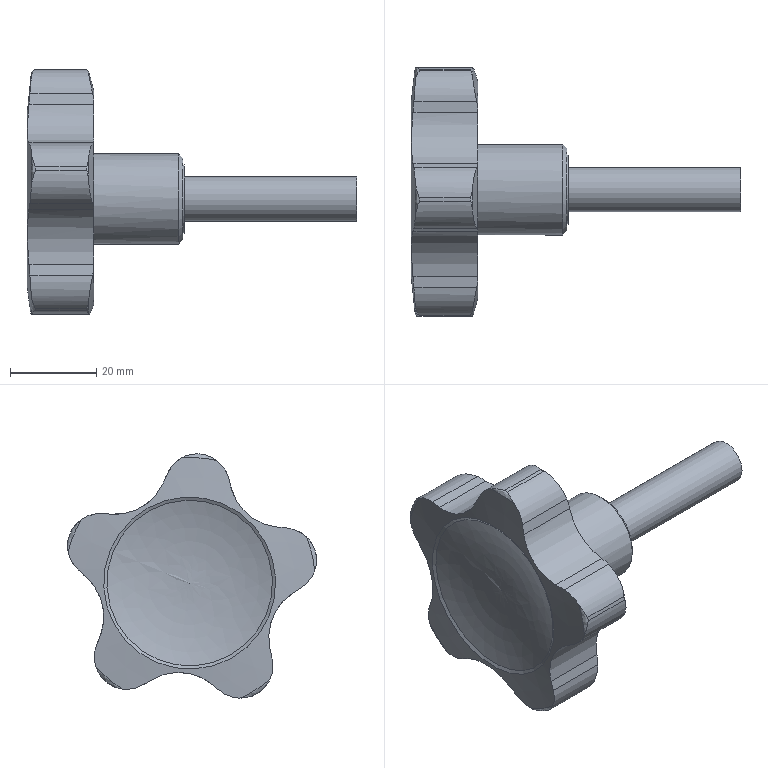Component | NX | 166552_X_T | 2 solids | 61 faces | volume 37139 mm3 | cylinder 24 | plane 15 | cone 10 | torus 10 | spline 2 | commonest cylinder face diameters 15 x10 60 x5 24.333 x5 21 x1 16 x1 8.376 x1 10.3 x1